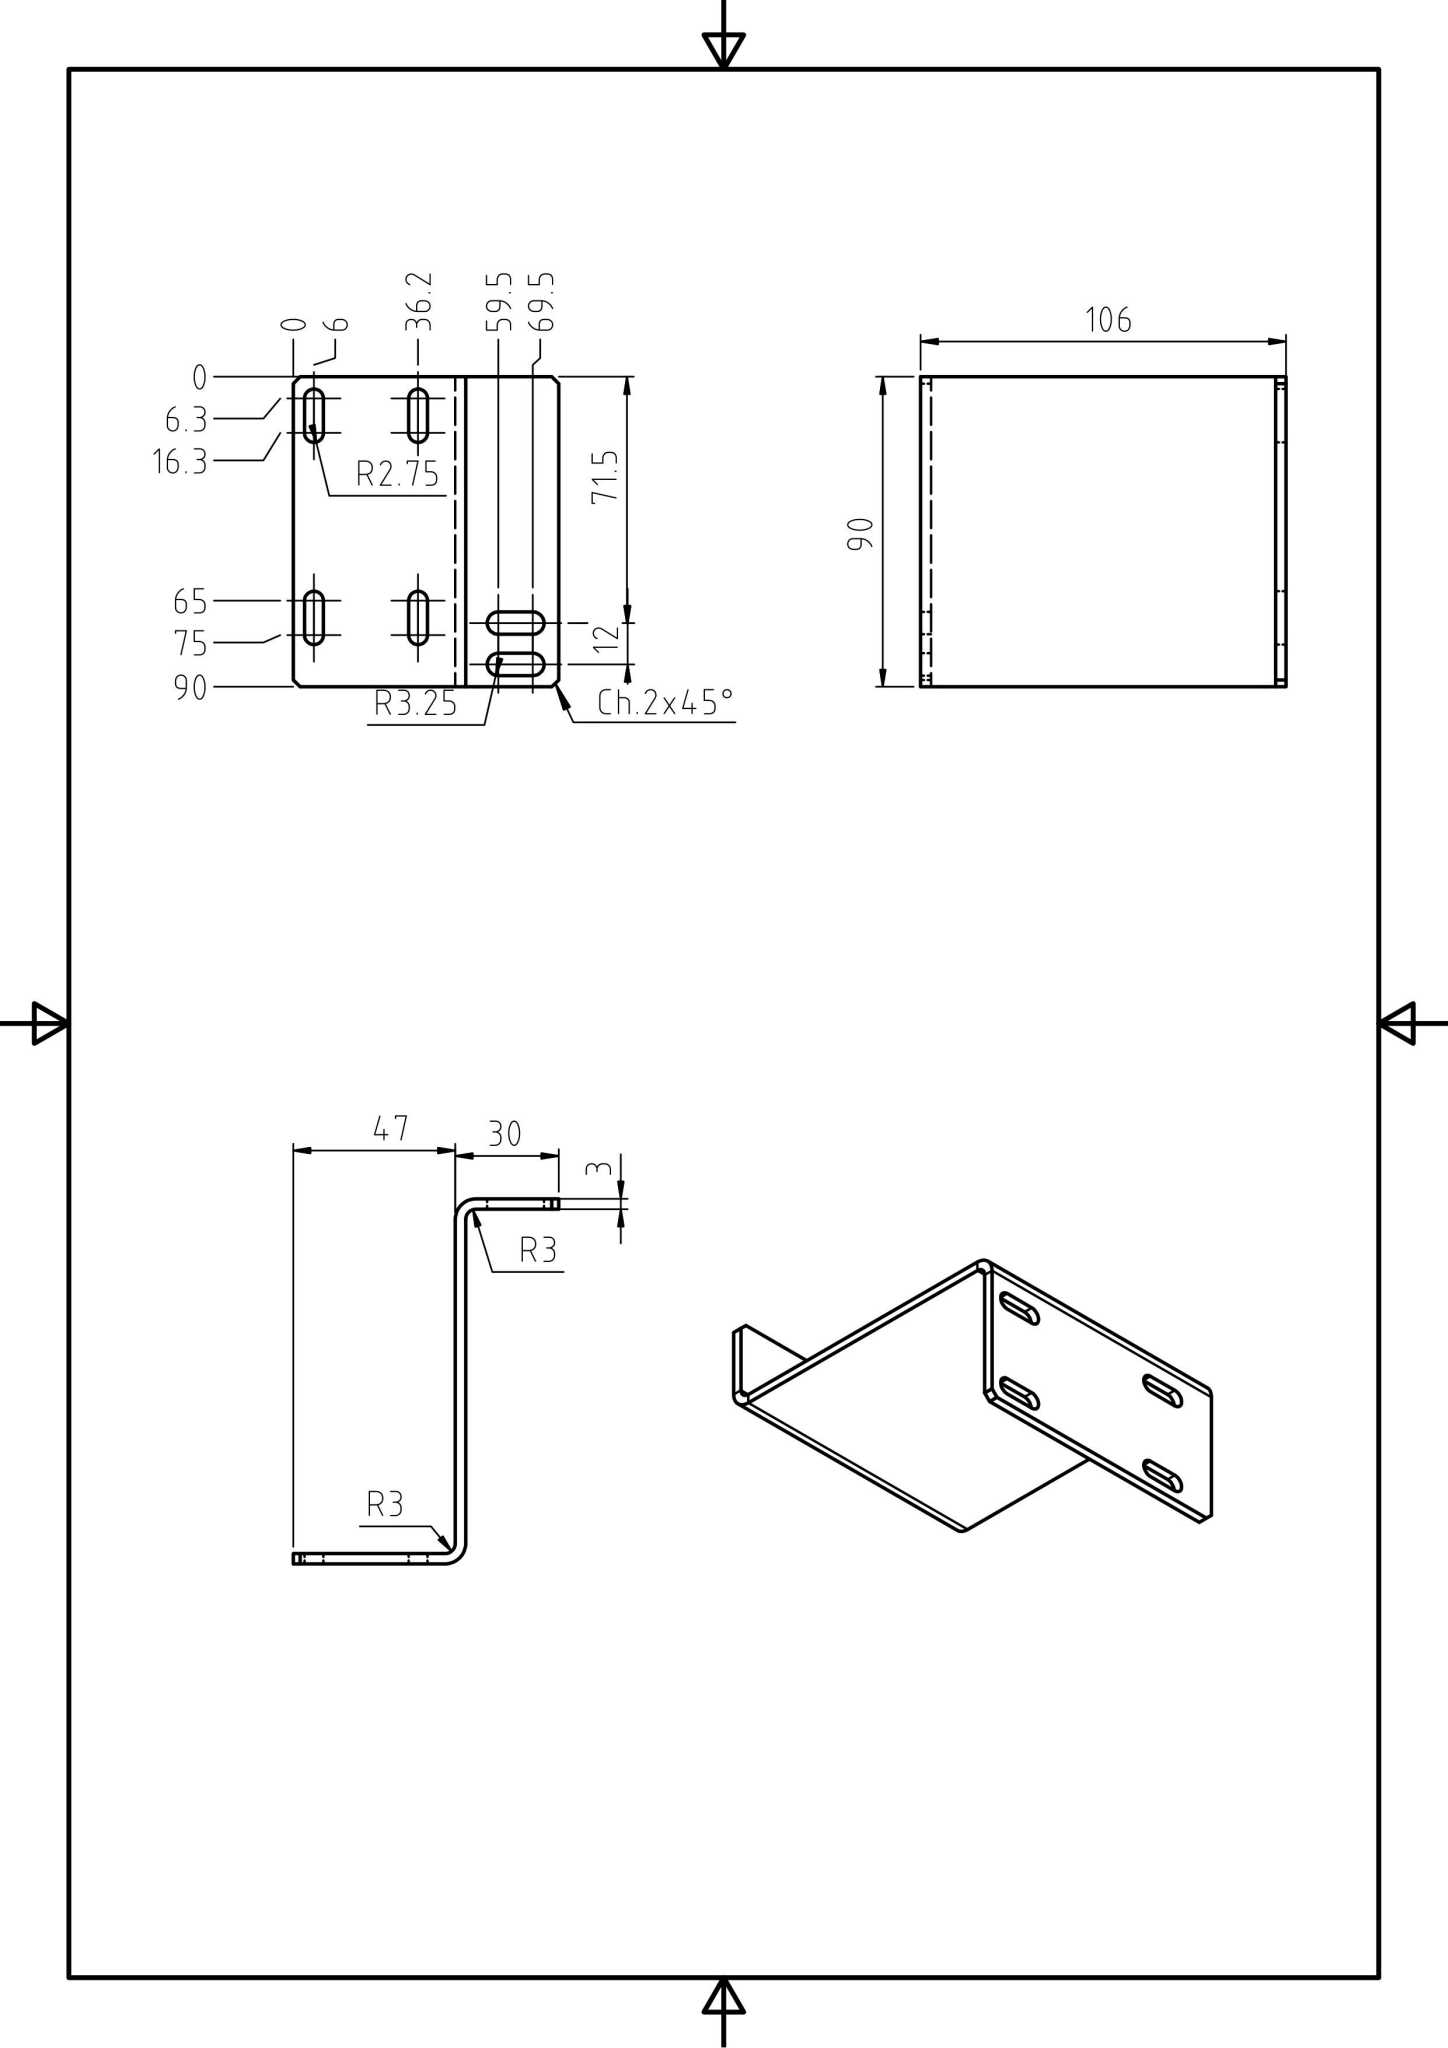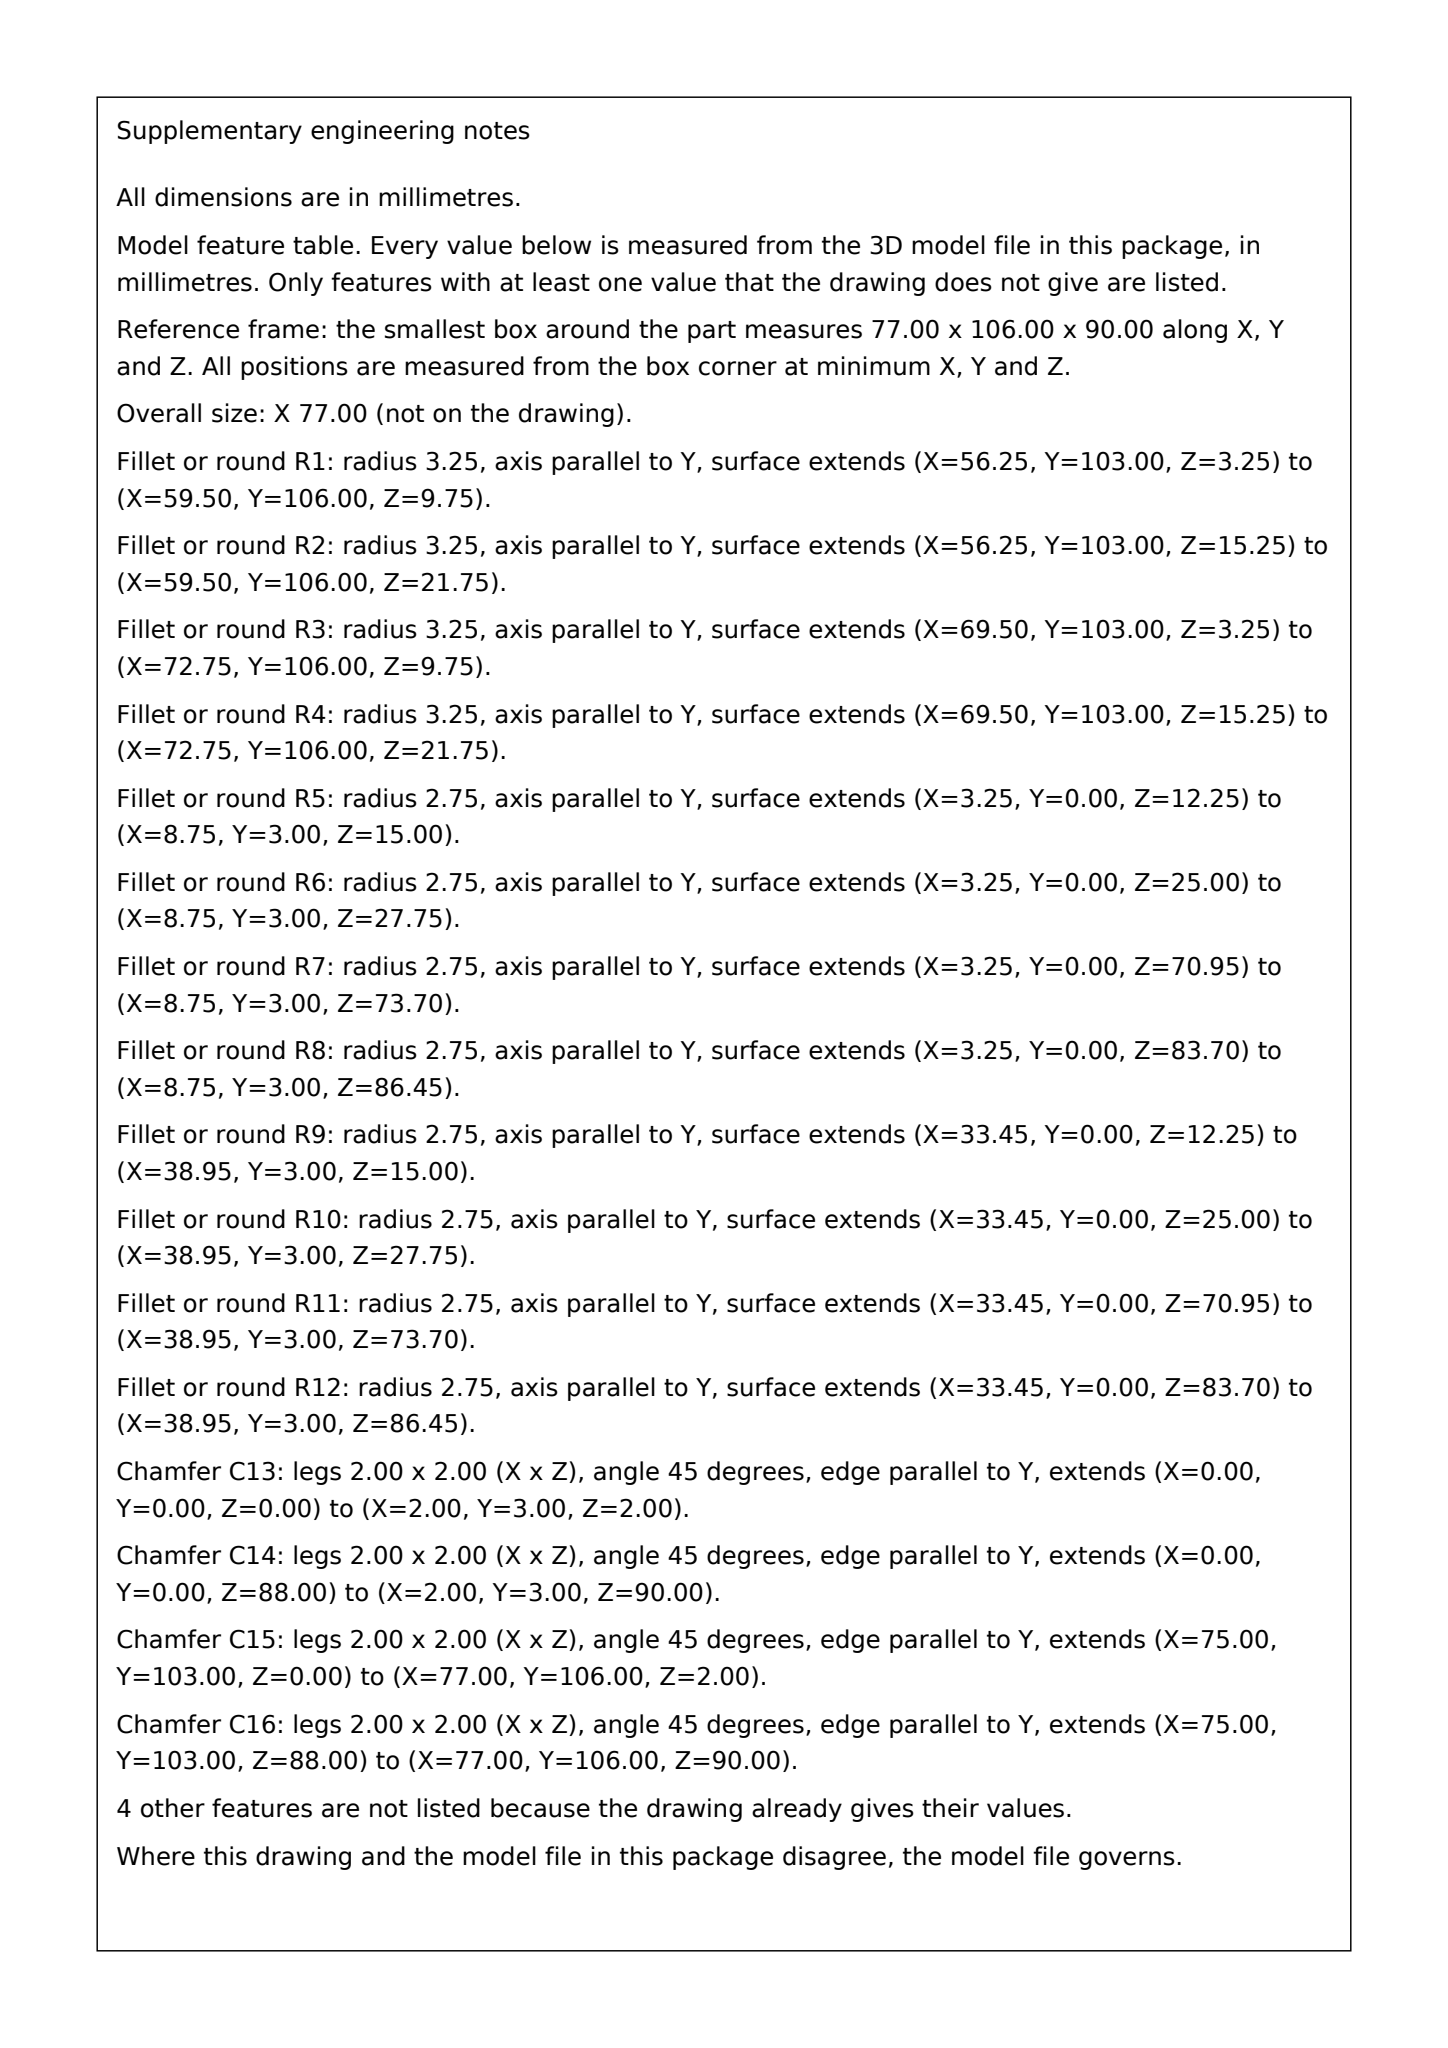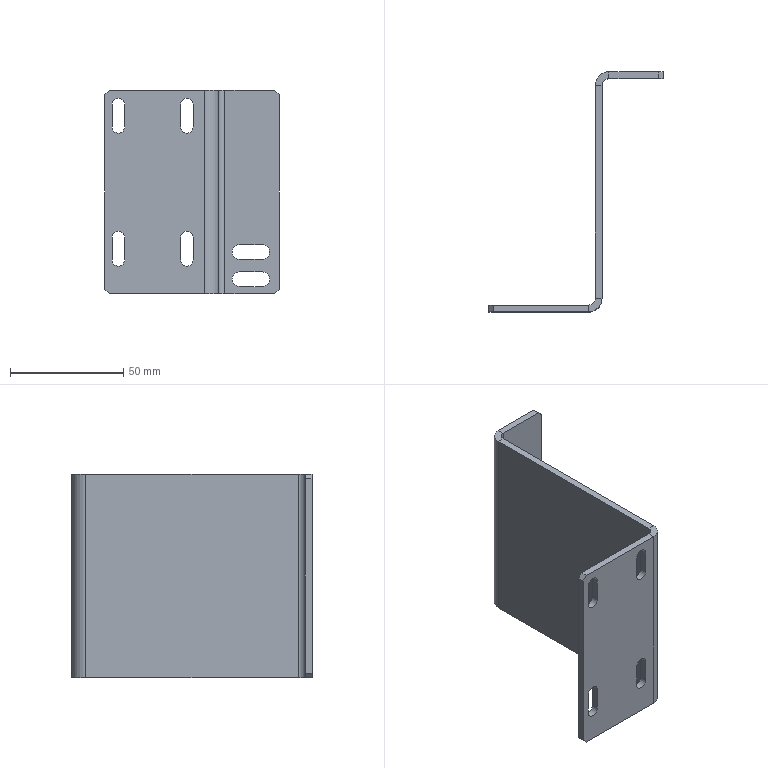Part | SolidWorks | mm | 1 solid | 50 faces | box 77 x 106 x 90 mm | volume 45999 mm3 | plane 34 | cylinder 16 | commonest cylinder face diameters 5.5 x8 6.5 x4 12 x2 6 x2